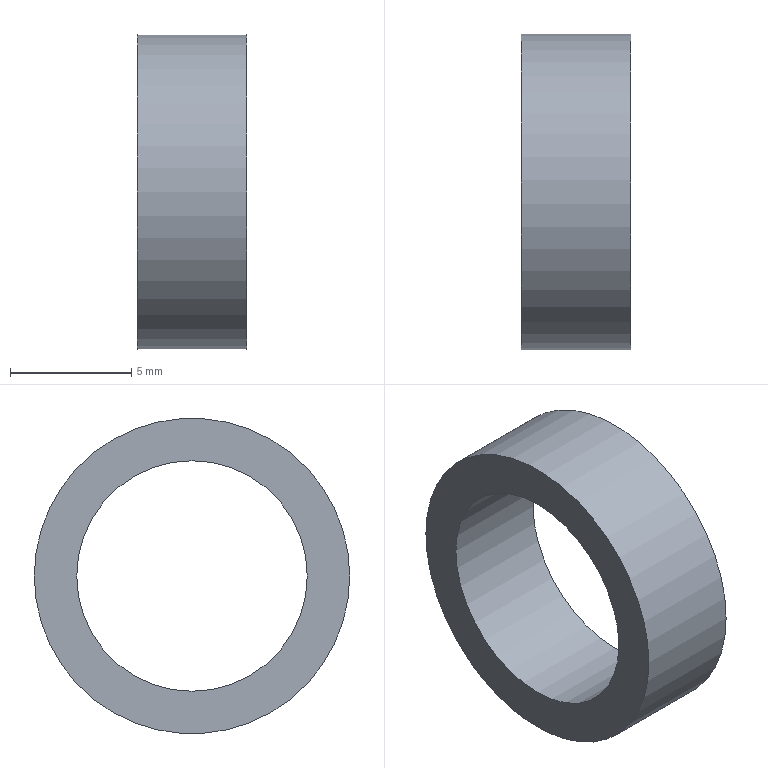Component | NX | WASHER | 1 solid | 4 faces | box 4.5 x 13 x 13 mm | volume 278 mm3 | cylinder 2 | plane 2 | commonest cylinder face diameters 13 x1 9.5 x1
STEP:
#1=CARTESIAN_POINT('',(0.,0.,0.));
#2=DIRECTION('',(0.,0.,1.));
#3=DIRECTION('',(1.,0.,0.));
#4=AXIS2_PLACEMENT_3D('',#1,#2,#3);
#5=CARTESIAN_POINT('',(-155.,-6.5,255.5));
#6=VERTEX_POINT('',#5);
#7=CARTESIAN_POINT('',(-155.,-0.,255.5));
#8=DIRECTION('',(-1.,0.,0.));
#9=DIRECTION('',(0.,-1.,0.));
#10=AXIS2_PLACEMENT_3D('',#7,#8,#9);
#11=CIRCLE('',#10,6.5);
#12=CARTESIAN_POINT('',(-155.,-0.,255.5));
#13=DIRECTION('',(1.,0.,0.));
#14=DIRECTION('',(0.,1.,0.));
#15=AXIS2_PLACEMENT_3D('',#12,#13,#14);
#16=CYLINDRICAL_SURFACE('',#15,6.5);
#17=CARTESIAN_POINT('',(9.425,0.));
#18=DIRECTION('',(-1.,0.));
#19=VECTOR('',#18,1.);
#20=LINE('',#17,#19);
#21=(GEOMETRIC_REPRESENTATION_CONTEXT(2)PARAMETRIC_REPRESENTATION_CONTEXT()REPRESENTATION_CONTEXT('',''));
#22=DEFINITIONAL_REPRESENTATION('',(#20),#21);
#23=PCURVE('',#16,#22);
#24=CARTESIAN_POINT('',(-155.,-0.,255.5));
#25=DIRECTION('',(-1.,0.,0.));
#26=DIRECTION('',(0.,-1.,0.));
#27=AXIS2_PLACEMENT_3D('',#24,#25,#26);
#28=PLANE('',#27);
#29=CARTESIAN_POINT('',(0.,0.));
#30=DIRECTION('',(1.,0.));
#31=AXIS2_PLACEMENT_2D('',#29,#30);
#32=CIRCLE('',#31,6.5);
#33=(GEOMETRIC_REPRESENTATION_CONTEXT(2)PARAMETRIC_REPRESENTATION_CONTEXT()REPRESENTATION_CONTEXT('',''));
#34=DEFINITIONAL_REPRESENTATION('',(#32),#33);
#35=PCURVE('',#28,#34);
#36=SURFACE_CURVE('',#11,(#23,#35),.PCURVE_S1.);
#37=EDGE_CURVE('',#6,#6,#36,.T.);
#38=ORIENTED_EDGE('',*,*,#37,.F.);
#39=CARTESIAN_POINT('',(-150.5,-6.5,255.5));
#40=VERTEX_POINT('',#39);
#41=CARTESIAN_POINT('',(-155.,-6.5,255.5));
#42=CARTESIAN_POINT('',(-150.5,-6.5,255.5));
#43=B_SPLINE_CURVE_WITH_KNOTS('',1,(#41,#42),.UNSPECIFIED.,.F.,.F.,(2,2),(0.,4.5),.PIECEWISE_BEZIER_KNOTS.);
#44=CARTESIAN_POINT('',(9.425,0.));
#45=DIRECTION('',(0.,1.));
#46=VECTOR('',#45,1.);
#47=LINE('',#44,#46);
#48=(GEOMETRIC_REPRESENTATION_CONTEXT(2)PARAMETRIC_REPRESENTATION_CONTEXT()REPRESENTATION_CONTEXT('',''));
#49=DEFINITIONAL_REPRESENTATION('',(#47),#48);
#50=PCURVE('',#16,#49);
#51=CARTESIAN_POINT('',(3.142,0.));
#52=DIRECTION('',(0.,1.));
#53=VECTOR('',#52,1.);
#54=LINE('',#51,#53);
#55=(GEOMETRIC_REPRESENTATION_CONTEXT(2)PARAMETRIC_REPRESENTATION_CONTEXT()REPRESENTATION_CONTEXT('',''));
#56=DEFINITIONAL_REPRESENTATION('',(#54),#55);
#57=PCURVE('',#16,#56);
#58=SEAM_CURVE('',#43,(#50,#57),.PCURVE_S1.);
#59=EDGE_CURVE('',#6,#40,#58,.T.);
#60=ORIENTED_EDGE('',*,*,#59,.T.);
#61=CARTESIAN_POINT('',(-150.5,-0.,255.5));
#62=DIRECTION('',(-1.,0.,0.));
#63=DIRECTION('',(0.,-1.,0.));
#64=AXIS2_PLACEMENT_3D('',#61,#62,#63);
#65=CIRCLE('',#64,6.5);
#66=CARTESIAN_POINT('',(9.425,4.5));
#67=DIRECTION('',(-1.,0.));
#68=VECTOR('',#67,1.);
#69=LINE('',#66,#68);
#70=(GEOMETRIC_REPRESENTATION_CONTEXT(2)PARAMETRIC_REPRESENTATION_CONTEXT()REPRESENTATION_CONTEXT('',''));
#71=DEFINITIONAL_REPRESENTATION('',(#69),#70);
#72=PCURVE('',#16,#71);
#73=CARTESIAN_POINT('',(-150.5,-0.,255.5));
#74=DIRECTION('',(-1.,0.,0.));
#75=DIRECTION('',(0.,-1.,0.));
#76=AXIS2_PLACEMENT_3D('',#73,#74,#75);
#77=PLANE('',#76);
#78=CARTESIAN_POINT('',(0.,0.));
#79=DIRECTION('',(1.,0.));
#80=AXIS2_PLACEMENT_2D('',#78,#79);
#81=CIRCLE('',#80,6.5);
#82=(GEOMETRIC_REPRESENTATION_CONTEXT(2)PARAMETRIC_REPRESENTATION_CONTEXT()REPRESENTATION_CONTEXT('',''));
#83=DEFINITIONAL_REPRESENTATION('',(#81),#82);
#84=PCURVE('',#77,#83);
#85=SURFACE_CURVE('',#65,(#72,#84),.PCURVE_S1.);
#86=EDGE_CURVE('',#40,#40,#85,.T.);
#87=ORIENTED_EDGE('',*,*,#86,.T.);
#88=ORIENTED_EDGE('',*,*,#59,.F.);
#89=EDGE_LOOP('',(#38,#60,#87,#88));
#90=FACE_BOUND('',#89,.T.);
#91=ADVANCED_FACE('',(#90),#16,.T.);
#92=CARTESIAN_POINT('',(-155.,-4.75,255.5));
#93=VERTEX_POINT('',#92);
#94=CARTESIAN_POINT('',(-155.,-0.,255.5));
#95=DIRECTION('',(-1.,0.,0.));
#96=DIRECTION('',(0.,-1.,0.));
#97=AXIS2_PLACEMENT_3D('',#94,#95,#96);
#98=CIRCLE('',#97,4.75);
#99=CARTESIAN_POINT('',(-155.,-0.,255.5));
#100=DIRECTION('',(1.,0.,0.));
#101=DIRECTION('',(0.,1.,0.));
#102=AXIS2_PLACEMENT_3D('',#99,#100,#101);
#103=CYLINDRICAL_SURFACE('',#102,4.75);
#104=CARTESIAN_POINT('',(9.425,0.));
#105=DIRECTION('',(-1.,0.));
#106=VECTOR('',#105,1.);
#107=LINE('',#104,#106);
#108=(GEOMETRIC_REPRESENTATION_CONTEXT(2)PARAMETRIC_REPRESENTATION_CONTEXT()REPRESENTATION_CONTEXT('',''));
#109=DEFINITIONAL_REPRESENTATION('',(#107),#108);
#110=PCURVE('',#103,#109);
#111=CARTESIAN_POINT('',(0.,0.));
#112=DIRECTION('',(1.,0.));
#113=AXIS2_PLACEMENT_2D('',#111,#112);
#114=CIRCLE('',#113,4.75);
#115=(GEOMETRIC_REPRESENTATION_CONTEXT(2)PARAMETRIC_REPRESENTATION_CONTEXT()REPRESENTATION_CONTEXT('',''));
#116=DEFINITIONAL_REPRESENTATION('',(#114),#115);
#117=PCURVE('',#28,#116);
#118=SURFACE_CURVE('',#98,(#110,#117),.PCURVE_S1.);
#119=EDGE_CURVE('',#93,#93,#118,.T.);
#120=ORIENTED_EDGE('',*,*,#119,.F.);
#121=CARTESIAN_POINT('',(-150.5,-4.75,255.5));
#122=VERTEX_POINT('',#121);
#123=CARTESIAN_POINT('',(-155.,-4.75,255.5));
#124=CARTESIAN_POINT('',(-150.5,-4.75,255.5));
#125=B_SPLINE_CURVE_WITH_KNOTS('',1,(#123,#124),.UNSPECIFIED.,.F.,.F.,(2,2),(0.,4.5),.PIECEWISE_BEZIER_KNOTS.);
#126=CARTESIAN_POINT('',(9.425,0.));
#127=DIRECTION('',(0.,1.));
#128=VECTOR('',#127,1.);
#129=LINE('',#126,#128);
#130=(GEOMETRIC_REPRESENTATION_CONTEXT(2)PARAMETRIC_REPRESENTATION_CONTEXT()REPRESENTATION_CONTEXT('',''));
#131=DEFINITIONAL_REPRESENTATION('',(#129),#130);
#132=PCURVE('',#103,#131);
#133=CARTESIAN_POINT('',(3.142,0.));
#134=DIRECTION('',(0.,1.));
#135=VECTOR('',#134,1.);
#136=LINE('',#133,#135);
#137=(GEOMETRIC_REPRESENTATION_CONTEXT(2)PARAMETRIC_REPRESENTATION_CONTEXT()REPRESENTATION_CONTEXT('',''));
#138=DEFINITIONAL_REPRESENTATION('',(#136),#137);
#139=PCURVE('',#103,#138);
#140=SEAM_CURVE('',#125,(#132,#139),.PCURVE_S1.);
#141=EDGE_CURVE('',#93,#122,#140,.T.);
#142=ORIENTED_EDGE('',*,*,#141,.T.);
#143=CARTESIAN_POINT('',(-150.5,-0.,255.5));
#144=DIRECTION('',(-1.,0.,0.));
#145=DIRECTION('',(0.,-1.,0.));
#146=AXIS2_PLACEMENT_3D('',#143,#144,#145);
#147=CIRCLE('',#146,4.75);
#148=CARTESIAN_POINT('',(9.425,4.5));
#149=DIRECTION('',(-1.,0.));
#150=VECTOR('',#149,1.);
#151=LINE('',#148,#150);
#152=(GEOMETRIC_REPRESENTATION_CONTEXT(2)PARAMETRIC_REPRESENTATION_CONTEXT()REPRESENTATION_CONTEXT('',''));
#153=DEFINITIONAL_REPRESENTATION('',(#151),#152);
#154=PCURVE('',#103,#153);
#155=CARTESIAN_POINT('',(0.,0.));
#156=DIRECTION('',(1.,0.));
#157=AXIS2_PLACEMENT_2D('',#155,#156);
#158=CIRCLE('',#157,4.75);
#159=(GEOMETRIC_REPRESENTATION_CONTEXT(2)PARAMETRIC_REPRESENTATION_CONTEXT()REPRESENTATION_CONTEXT('',''));
#160=DEFINITIONAL_REPRESENTATION('',(#158),#159);
#161=PCURVE('',#77,#160);
#162=SURFACE_CURVE('',#147,(#154,#161),.PCURVE_S1.);
#163=EDGE_CURVE('',#122,#122,#162,.T.);
#164=ORIENTED_EDGE('',*,*,#163,.T.);
#165=ORIENTED_EDGE('',*,*,#141,.F.);
#166=EDGE_LOOP('',(#120,#142,#164,#165));
#167=FACE_BOUND('',#166,.F.);
#168=ADVANCED_FACE('',(#167),#103,.F.);
#169=ORIENTED_EDGE('',*,*,#37,.T.);
#170=EDGE_LOOP('',(#169));
#171=FACE_BOUND('',#170,.T.);
#172=ORIENTED_EDGE('',*,*,#119,.F.);
#173=EDGE_LOOP('',(#172));
#174=FACE_BOUND('',#173,.T.);
#175=ADVANCED_FACE('',(#171,#174),#28,.T.);
#176=ORIENTED_EDGE('',*,*,#86,.F.);
#177=EDGE_LOOP('',(#176));
#178=FACE_BOUND('',#177,.T.);
#179=ORIENTED_EDGE('',*,*,#163,.T.);
#180=EDGE_LOOP('',(#179));
#181=FACE_BOUND('',#180,.T.);
#182=ADVANCED_FACE('',(#178,#181),#77,.F.);
#183=CLOSED_SHELL('',(#91,#168,#175,#182));
#184=MANIFOLD_SOLID_BREP('',#183);
#185=(LENGTH_UNIT()NAMED_UNIT(*)SI_UNIT(.MILLI.,.METRE.));
#186=UNCERTAINTY_MEASURE_WITH_UNIT(LENGTH_MEASURE(0.00001),#185,'','');
#187=(NAMED_UNIT(*)PLANE_ANGLE_UNIT()SI_UNIT($,.RADIAN.));
#188=(NAMED_UNIT(*)SI_UNIT($,.STERADIAN.)SOLID_ANGLE_UNIT());
#189=(GEOMETRIC_REPRESENTATION_CONTEXT(3)GLOBAL_UNCERTAINTY_ASSIGNED_CONTEXT((#186))GLOBAL_UNIT_ASSIGNED_CONTEXT((#185,#187,#188))REPRESENTATION_CONTEXT('',''));
#190=ADVANCED_BREP_SHAPE_REPRESENTATION('',(#4,#184),#189);